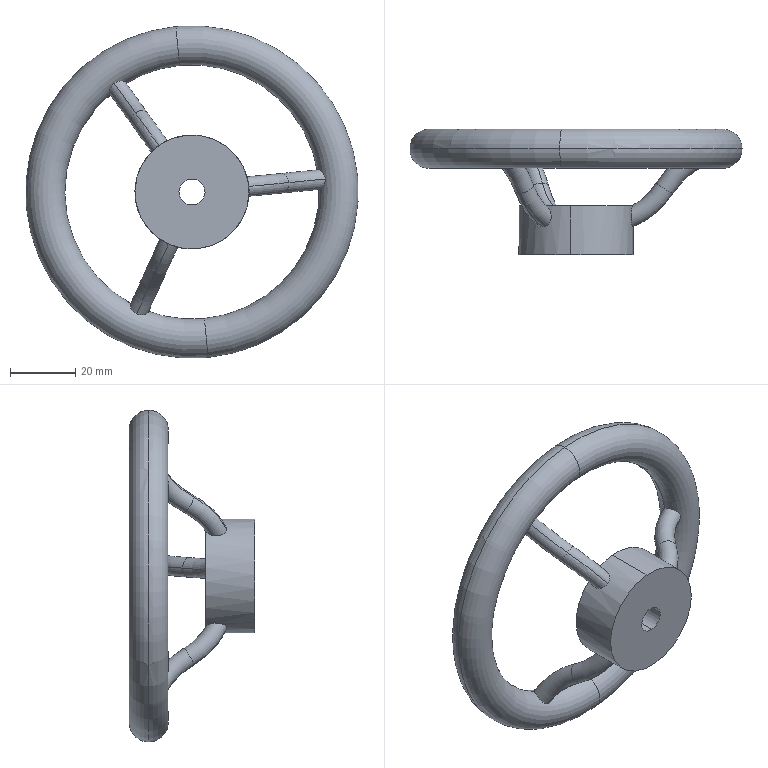Component | SolidWorks | Handle1-1-1 | 1 solid | 22 faces | volume 48149 mm3 | torus 16 | cylinder 4 | plane 2 | commonest cylinder face diameters 8 x2 35 x2